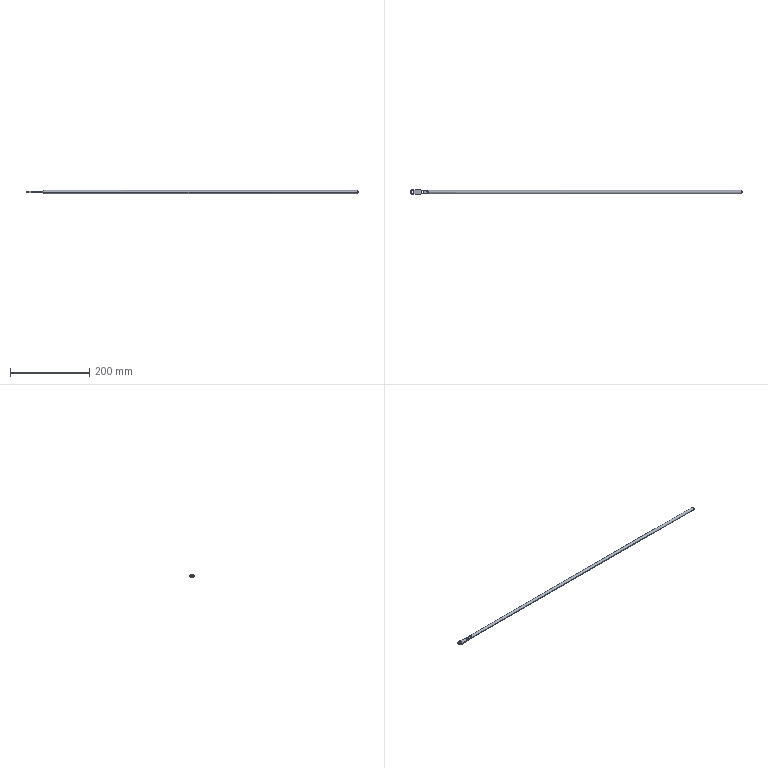Component | SolidWorks | FrontDoorAssembly-1_FrontDoorLowerLockRod-1 | 1 solid | 20 faces | box 837.5 x 13 x 8 mm | volume 41039 mm3 | plane 11 | cylinder 7 | cone 2 | commonest cylinder face diameters 6.5 x4 8 x2 13 x1
build123d program:
from build123d import *

# Parameters (mm, degrees)
SKETCH1_R           = 4
BOSS_EXTRUDE1_DEPTH = 837.5
CUT_EXTRUDE1_DEPTH  = 5
SKETCH3_W           = 42
SKETCH3_H           = 2.024
CUT_EXTRUDE2_DEPTH  = 10
BOSS_EXTRUDE2_DEPTH = 3
CUT_EXTRUDE3_DEPTH  = 3
SKETCH6_R           = 3.25
CUT_EXTRUDE4_DEPTH  = 3
CHAMFER1_SIZE       = 1.5


with BuildPart() as part:
    # Sketch1 → Boss-Extrude1 (new body)
    with BuildSketch(Plane(origin=(0, 0, 0), x_dir=(0, 0, -1), z_dir=(1, 0, 0))):
        Circle(SKETCH1_R)
    extrude(amount=-BOSS_EXTRUDE1_DEPTH)

    # Sketch2 → Cut-Extrude1 (cut, symmetric)
    with BuildSketch(Plane.XY):
        Polygon((-42, 1.5), (-45.678, 4), (-42, 4), (0, 4), (0, 1.5), align=None)
        Polygon((-45.678, -4), (-42, -4), (0, -4), (0, -1.5), (-42, -1.5), align=None)
    extrude(amount=CUT_EXTRUDE1_DEPTH, both=True, mode=Mode.SUBTRACT)

    # Sketch3 → Cut-Extrude2 (cut)
    with BuildSketch(Plane(origin=(0, 1.5, 0), x_dir=(1, 0, 0), z_dir=(0, 1, 0))):
        with Locations((-21, 2.988)):
            Rectangle(SKETCH3_W, SKETCH3_H)
        with Locations((-21, -2.988)):
            Rectangle(SKETCH3_W, SKETCH3_H)
    extrude(amount=-CUT_EXTRUDE2_DEPTH, mode=Mode.SUBTRACT)

    # Sketch4 → Boss-Extrude2 (add)
    with BuildSketch(Plane(origin=(0, 1.5, 0), x_dir=(1, 0, 0), z_dir=(0, 1, 0))):
        with BuildLine():
            Line((-42, -4), (-42, 4))
            Line((-42, 4), (-7.386, 6.439))
            ThreePointArc((-7.386, 6.439), (0, 0), (-7.386, -6.439))
            Line((-7.386, -6.439), (-42, -4))
        make_face()
    extrude(amount=-BOSS_EXTRUDE2_DEPTH)

    # Sketch5 → Cut-Extrude3 (cut)
    with BuildSketch(Plane(origin=(0, 1.5, 0), x_dir=(1, 0, 0), z_dir=(0, 1, 0))):
        with BuildLine():
            Line((-0.8017, 3.127), (2.344, 3.127))
            Line((2.344, 3.127), (2.344, -3.404))
            Line((2.344, -3.404), (-0.9628, -3.404))
            ThreePointArc((-0.9628, -3.404), (-0.001977, -0.1603), (-0.8017, 3.127))
        make_face()
    extrude(amount=-CUT_EXTRUDE3_DEPTH, mode=Mode.SUBTRACT)

    # Sketch6 → Cut-Extrude4 (cut)
    with BuildSketch(Plane(origin=(0, 1.5, 0), x_dir=(1, 0, 0), z_dir=(0, 1, 0))):
        with Locations(Location((-6, 0, 0), (0, 0, 180))):
            Circle(SKETCH6_R)
        with Locations(Location((-31, 0, 0), (0, 0, 180))):
            Circle(SKETCH6_R)
    extrude(amount=-CUT_EXTRUDE4_DEPTH, mode=Mode.SUBTRACT)

    # Chamfer1
    chamfer1_edges = [part.edges().sort_by_distance(p)[0] for p in [
        (-837.5, 0, 4),
    ]]
    chamfer(chamfer1_edges, length=CHAMFER1_SIZE)


solid = part.part

# Placed as in the assembly
solid = solid.moved(Location((30.814, -273.299, 374.754), (-90, 0, 180)))
STEP:
#1=COLOUR_RGB('',0.7922,0.8196,0.9333);
#2=FILL_AREA_STYLE_COLOUR('',#1);
#3=FILL_AREA_STYLE('',(#2));
#4=SURFACE_STYLE_FILL_AREA(#3);
#5=SURFACE_SIDE_STYLE('',(#4));
#6=SURFACE_STYLE_USAGE(.BOTH.,#5);
#7=PRESENTATION_STYLE_ASSIGNMENT((#6));
#8=CARTESIAN_POINT('',(34.186,-10.661,14.754));
#9=VERTEX_POINT('',#8);
#10=CARTESIAN_POINT('',(34.186,-10.858,14.754));
#11=VERTEX_POINT('',#10);
#12=CARTESIAN_POINT('',(34.186,-10.76,14.754));
#13=DIRECTION('',(1.,0.,-0.));
#14=DIRECTION('',(0.,-1.,0.));
#15=AXIS2_PLACEMENT_3D('',#12,#13,#14);
#16=CIRCLE('',#15,0.09843);
#17=EDGE_CURVE('',#9,#11,#16,.T.);
#18=ORIENTED_EDGE('',*,*,#17,.F.);
#19=CARTESIAN_POINT('',(34.127,-10.602,14.754));
#20=VERTEX_POINT('',#19);
#21=CARTESIAN_POINT('',(34.127,-10.602,14.754));
#22=DIRECTION('',(-0.7071,0.7071,0.));
#23=VECTOR('',#22,39.37);
#24=LINE('',#21,#23);
#25=EDGE_CURVE('',#9,#20,#24,.T.);
#26=ORIENTED_EDGE('',*,*,#25,.T.);
#27=CARTESIAN_POINT('',(34.127,-10.917,14.754));
#28=VERTEX_POINT('',#27);
#29=CARTESIAN_POINT('',(34.127,-10.76,14.754));
#30=DIRECTION('',(-1.,-0.,0.));
#31=DIRECTION('',(0.,-1.,0.));
#32=AXIS2_PLACEMENT_3D('',#29,#30,#31);
#33=CIRCLE('',#32,0.1575);
#34=EDGE_CURVE('',#28,#20,#33,.T.);
#35=ORIENTED_EDGE('',*,*,#34,.F.);
#36=CARTESIAN_POINT('',(34.127,-10.917,14.754));
#37=DIRECTION('',(-0.7071,-0.7071,0.));
#38=VECTOR('',#37,39.37);
#39=LINE('',#36,#38);
#40=EDGE_CURVE('',#11,#28,#39,.T.);
#41=ORIENTED_EDGE('',*,*,#40,.F.);
#42=EDGE_LOOP('',(#18,#26,#35,#41));
#43=FACE_OUTER_BOUND('',#42,.T.);
#44=CARTESIAN_POINT('',(34.127,-10.76,14.754));
#45=DIRECTION('',(-1.,-0.,0.));
#46=DIRECTION('',(0.,-1.,0.));
#47=AXIS2_PLACEMENT_3D('',#44,#45,#46);
#48=CONICAL_SURFACE('',#47,0.1575,0.7854);
#49=ADVANCED_FACE('',(#43),#48,.T.);
#50=CARTESIAN_POINT('',(2.306,-10.76,14.695));
#51=VERTEX_POINT('',#50);
#52=CARTESIAN_POINT('',(2.562,-10.76,14.695));
#53=VERTEX_POINT('',#52);
#54=CARTESIAN_POINT('',(2.434,-10.76,14.695));
#55=DIRECTION('',(0.,0.,1.));
#56=DIRECTION('',(1.,0.,0.));
#57=AXIS2_PLACEMENT_3D('',#54,#55,#56);
#58=CIRCLE('',#57,0.128);
#59=EDGE_CURVE('',#51,#53,#58,.T.);
#60=ORIENTED_EDGE('',*,*,#59,.F.);
#61=CARTESIAN_POINT('',(2.306,-10.76,14.813));
#62=VERTEX_POINT('',#61);
#63=CARTESIAN_POINT('',(2.306,-10.76,14.695));
#64=DIRECTION('',(0.,0.,1.));
#65=VECTOR('',#64,39.37);
#66=LINE('',#63,#65);
#67=EDGE_CURVE('',#51,#62,#66,.T.);
#68=ORIENTED_EDGE('',*,*,#67,.T.);
#69=CARTESIAN_POINT('',(2.562,-10.76,14.813));
#70=VERTEX_POINT('',#69);
#71=CARTESIAN_POINT('',(2.434,-10.76,14.813));
#72=DIRECTION('',(0.,0.,1.));
#73=DIRECTION('',(1.,0.,0.));
#74=AXIS2_PLACEMENT_3D('',#71,#72,#73);
#75=CIRCLE('',#74,0.128);
#76=EDGE_CURVE('',#62,#70,#75,.T.);
#77=ORIENTED_EDGE('',*,*,#76,.T.);
#78=CARTESIAN_POINT('',(2.562,-10.76,14.695));
#79=DIRECTION('',(0.,0.,1.));
#80=VECTOR('',#79,39.37);
#81=LINE('',#78,#80);
#82=EDGE_CURVE('',#53,#70,#81,.T.);
#83=ORIENTED_EDGE('',*,*,#82,.F.);
#84=EDGE_LOOP('',(#60,#68,#77,#83));
#85=FACE_OUTER_BOUND('',#84,.T.);
#86=CARTESIAN_POINT('',(2.434,-10.76,14.695));
#87=DIRECTION('',(0.,0.,1.));
#88=DIRECTION('',(1.,0.,0.));
#89=AXIS2_PLACEMENT_3D('',#86,#87,#88);
#90=CYLINDRICAL_SURFACE('',#89,0.128);
#91=ADVANCED_FACE('',(#85),#90,.F.);
#92=CARTESIAN_POINT('',(1.321,-10.76,14.695));
#93=VERTEX_POINT('',#92);
#94=CARTESIAN_POINT('',(1.577,-10.76,14.695));
#95=VERTEX_POINT('',#94);
#96=CARTESIAN_POINT('',(1.449,-10.76,14.695));
#97=DIRECTION('',(0.,0.,1.));
#98=DIRECTION('',(1.,0.,0.));
#99=AXIS2_PLACEMENT_3D('',#96,#97,#98);
#100=CIRCLE('',#99,0.128);
#101=EDGE_CURVE('',#93,#95,#100,.T.);
#102=ORIENTED_EDGE('',*,*,#101,.F.);
#103=CARTESIAN_POINT('',(1.321,-10.76,14.813));
#104=VERTEX_POINT('',#103);
#105=CARTESIAN_POINT('',(1.321,-10.76,14.695));
#106=DIRECTION('',(0.,0.,1.));
#107=VECTOR('',#106,39.37);
#108=LINE('',#105,#107);
#109=EDGE_CURVE('',#93,#104,#108,.T.);
#110=ORIENTED_EDGE('',*,*,#109,.T.);
#111=CARTESIAN_POINT('',(1.577,-10.76,14.813));
#112=VERTEX_POINT('',#111);
#113=CARTESIAN_POINT('',(1.449,-10.76,14.813));
#114=DIRECTION('',(0.,0.,1.));
#115=DIRECTION('',(1.,0.,0.));
#116=AXIS2_PLACEMENT_3D('',#113,#114,#115);
#117=CIRCLE('',#116,0.128);
#118=EDGE_CURVE('',#104,#112,#117,.T.);
#119=ORIENTED_EDGE('',*,*,#118,.T.);
#120=CARTESIAN_POINT('',(1.577,-10.76,14.695));
#121=DIRECTION('',(0.,0.,1.));
#122=VECTOR('',#121,39.37);
#123=LINE('',#120,#122);
#124=EDGE_CURVE('',#95,#112,#123,.T.);
#125=ORIENTED_EDGE('',*,*,#124,.F.);
#126=EDGE_LOOP('',(#102,#110,#119,#125));
#127=FACE_OUTER_BOUND('',#126,.T.);
#128=CARTESIAN_POINT('',(1.449,-10.76,14.695));
#129=DIRECTION('',(0.,0.,1.));
#130=DIRECTION('',(1.,0.,0.));
#131=AXIS2_PLACEMENT_3D('',#128,#129,#130);
#132=CYLINDRICAL_SURFACE('',#131,0.128);
#133=ADVANCED_FACE('',(#127),#132,.F.);
#134=ORIENTED_EDGE('',*,*,#34,.T.);
#135=CARTESIAN_POINT('',(2.867,-10.602,14.754));
#136=VERTEX_POINT('',#135);
#137=CARTESIAN_POINT('',(34.186,-10.602,14.754));
#138=DIRECTION('',(-1.,-0.,0.));
#139=VECTOR('',#138,39.37);
#140=LINE('',#137,#139);
#141=EDGE_CURVE('',#20,#136,#140,.T.);
#142=ORIENTED_EDGE('',*,*,#141,.T.);
#143=CARTESIAN_POINT('',(2.867,-10.614,14.813));
#144=VERTEX_POINT('',#143);
#145=CARTESIAN_POINT('',(2.867,-10.76,14.754));
#146=DIRECTION('',(-1.,-0.,0.));
#147=DIRECTION('',(0.,0.,-1.));
#148=AXIS2_PLACEMENT_3D('',#145,#146,#147);
#149=CIRCLE('',#148,0.1575);
#150=EDGE_CURVE('',#144,#136,#149,.T.);
#151=ORIENTED_EDGE('',*,*,#150,.F.);
#152=CARTESIAN_POINT('',(2.867,-10.906,14.813));
#153=VERTEX_POINT('',#152);
#154=CARTESIAN_POINT('',(2.867,-10.906,14.813));
#155=CARTESIAN_POINT('',(3.094,-10.843,14.968));
#156=CARTESIAN_POINT('',(3.094,-10.676,14.968));
#157=CARTESIAN_POINT('',(2.867,-10.614,14.813));
#158=(BOUNDED_CURVE()B_SPLINE_CURVE(3,(#154,#155,#156,#157),.UNSPECIFIED.,.F.,.F.)B_SPLINE_CURVE_WITH_KNOTS((4,4),(1.955,4.328),.UNSPECIFIED.)CURVE()GEOMETRIC_REPRESENTATION_ITEM()RATIONAL_B_SPLINE_CURVE((1.,0.5833,0.5833,1.))REPRESENTATION_ITEM(''));
#159=EDGE_CURVE('',#153,#144,#158,.T.);
#160=ORIENTED_EDGE('',*,*,#159,.F.);
#161=CARTESIAN_POINT('',(2.867,-10.917,14.754));
#162=VERTEX_POINT('',#161);
#163=CARTESIAN_POINT('',(2.867,-10.76,14.754));
#164=DIRECTION('',(-1.,-0.,0.));
#165=DIRECTION('',(0.,0.,-1.));
#166=AXIS2_PLACEMENT_3D('',#163,#164,#165);
#167=CIRCLE('',#166,0.1575);
#168=EDGE_CURVE('',#162,#153,#167,.T.);
#169=ORIENTED_EDGE('',*,*,#168,.F.);
#170=CARTESIAN_POINT('',(34.186,-10.917,14.754));
#171=DIRECTION('',(-1.,-0.,0.));
#172=VECTOR('',#171,39.37);
#173=LINE('',#170,#172);
#174=EDGE_CURVE('',#28,#162,#173,.T.);
#175=ORIENTED_EDGE('',*,*,#174,.F.);
#176=EDGE_LOOP('',(#134,#142,#151,#160,#169,#175));
#177=FACE_OUTER_BOUND('',#176,.T.);
#178=CARTESIAN_POINT('',(34.186,-10.76,14.754));
#179=DIRECTION('',(-1.,-0.,0.));
#180=DIRECTION('',(0.,-1.,0.));
#181=AXIS2_PLACEMENT_3D('',#178,#179,#180);
#182=CYLINDRICAL_SURFACE('',#181,0.1575);
#183=ADVANCED_FACE('',(#177),#182,.T.);
#184=ORIENTED_EDGE('',*,*,#141,.F.);
#185=CARTESIAN_POINT('',(34.127,-10.76,14.754));
#186=DIRECTION('',(-1.,-0.,0.));
#187=DIRECTION('',(0.,-1.,0.));
#188=AXIS2_PLACEMENT_3D('',#185,#186,#187);
#189=CIRCLE('',#188,0.1575);
#190=EDGE_CURVE('',#20,#28,#189,.T.);
#191=ORIENTED_EDGE('',*,*,#190,.T.);
#192=ORIENTED_EDGE('',*,*,#174,.T.);
#193=CARTESIAN_POINT('',(2.867,-10.906,14.695));
#194=VERTEX_POINT('',#193);
#195=CARTESIAN_POINT('',(2.867,-10.76,14.754));
#196=DIRECTION('',(-1.,-0.,0.));
#197=DIRECTION('',(0.,-0.,-1.));
#198=AXIS2_PLACEMENT_3D('',#195,#196,#197);
#199=CIRCLE('',#198,0.1575);
#200=EDGE_CURVE('',#194,#162,#199,.T.);
#201=ORIENTED_EDGE('',*,*,#200,.F.);
#202=CARTESIAN_POINT('',(2.867,-10.614,14.695));
#203=VERTEX_POINT('',#202);
#204=CARTESIAN_POINT('',(2.867,-10.614,14.695));
#205=CARTESIAN_POINT('',(3.094,-10.676,14.54));
#206=CARTESIAN_POINT('',(3.094,-10.843,14.54));
#207=CARTESIAN_POINT('',(2.867,-10.906,14.695));
#208=(BOUNDED_CURVE()B_SPLINE_CURVE(3,(#204,#205,#206,#207),.UNSPECIFIED.,.F.,.F.)B_SPLINE_CURVE_WITH_KNOTS((4,4),(1.955,4.328),.UNSPECIFIED.)CURVE()GEOMETRIC_REPRESENTATION_ITEM()RATIONAL_B_SPLINE_CURVE((1.,0.5833,0.5833,1.))REPRESENTATION_ITEM(''));
#209=EDGE_CURVE('',#203,#194,#208,.T.);
#210=ORIENTED_EDGE('',*,*,#209,.F.);
#211=CARTESIAN_POINT('',(2.867,-10.76,14.754));
#212=DIRECTION('',(-1.,-0.,0.));
#213=DIRECTION('',(0.,-0.,-1.));
#214=AXIS2_PLACEMENT_3D('',#211,#212,#213);
#215=CIRCLE('',#214,0.1575);
#216=EDGE_CURVE('',#136,#203,#215,.T.);
#217=ORIENTED_EDGE('',*,*,#216,.F.);
#218=EDGE_LOOP('',(#184,#191,#192,#201,#210,#217));
#219=FACE_OUTER_BOUND('',#218,.T.);
#220=CARTESIAN_POINT('',(34.186,-10.76,14.754));
#221=DIRECTION('',(-1.,-0.,0.));
#222=DIRECTION('',(0.,-1.,0.));
#223=AXIS2_PLACEMENT_3D('',#220,#221,#222);
#224=CYLINDRICAL_SURFACE('',#223,0.1575);
#225=ADVANCED_FACE('',(#219),#224,.T.);
#226=CARTESIAN_POINT('',(34.186,-10.76,14.754));
#227=DIRECTION('',(1.,0.,-0.));
#228=DIRECTION('',(0.,-1.,0.));
#229=AXIS2_PLACEMENT_3D('',#226,#227,#228);
#230=CIRCLE('',#229,0.09843);
#231=EDGE_CURVE('',#11,#9,#230,.T.);
#232=ORIENTED_EDGE('',*,*,#231,.T.);
#233=ORIENTED_EDGE('',*,*,#17,.T.);
#234=EDGE_LOOP('',(#232,#233));
#235=FACE_OUTER_BOUND('',#234,.T.);
#236=CARTESIAN_POINT('',(34.186,-10.76,14.754));
#237=DIRECTION('',(-1.,-0.,0.));
#238=DIRECTION('',(0.,-1.,-0.));
#239=AXIS2_PLACEMENT_3D('',#236,#237,#238);
#240=PLANE('',#239);
#241=ADVANCED_FACE('',(#235),#240,.F.);
#242=CARTESIAN_POINT('',(2.434,-10.76,14.813));
#243=DIRECTION('',(0.,0.,1.));
#244=DIRECTION('',(1.,0.,0.));
#245=AXIS2_PLACEMENT_3D('',#242,#243,#244);
#246=CIRCLE('',#245,0.128);
#247=EDGE_CURVE('',#70,#62,#246,.T.);
#248=ORIENTED_EDGE('',*,*,#247,.F.);
#249=ORIENTED_EDGE('',*,*,#76,.F.);
#250=EDGE_LOOP('',(#248,#249));
#251=FACE_BOUND('',#250,.T.);
#252=CARTESIAN_POINT('',(1.449,-10.76,14.813));
#253=DIRECTION('',(0.,0.,1.));
#254=DIRECTION('',(1.,0.,0.));
#255=AXIS2_PLACEMENT_3D('',#252,#253,#254);
#256=CIRCLE('',#255,0.128);
#257=EDGE_CURVE('',#112,#104,#256,.T.);
#258=ORIENTED_EDGE('',*,*,#257,.F.);
#259=ORIENTED_EDGE('',*,*,#118,.F.);
#260=EDGE_LOOP('',(#258,#259));
#261=FACE_BOUND('',#260,.T.);
#262=CARTESIAN_POINT('',(2.867,-10.602,14.813));
#263=VERTEX_POINT('',#262);
#264=CARTESIAN_POINT('',(1.504,-10.506,14.813));
#265=VERTEX_POINT('',#264);
#266=CARTESIAN_POINT('',(2.867,-10.602,14.813));
#267=DIRECTION('',(-0.9975,0.0703,0.));
#268=VECTOR('',#267,39.37);
#269=LINE('',#266,#268);
#270=EDGE_CURVE('',#263,#265,#269,.T.);
#271=ORIENTED_EDGE('',*,*,#270,.T.);
#272=CARTESIAN_POINT('',(1.504,-11.013,14.813));
#273=VERTEX_POINT('',#272);
#274=CARTESIAN_POINT('',(1.469,-10.76,14.813));
#275=DIRECTION('',(0.,0.,1.));
#276=DIRECTION('',(1.,0.,0.));
#277=AXIS2_PLACEMENT_3D('',#274,#275,#276);
#278=CIRCLE('',#277,0.2559);
#279=EDGE_CURVE('',#265,#273,#278,.T.);
#280=ORIENTED_EDGE('',*,*,#279,.T.);
#281=CARTESIAN_POINT('',(2.867,-10.917,14.813));
#282=VERTEX_POINT('',#281);
#283=CARTESIAN_POINT('',(2.867,-10.917,14.813));
#284=DIRECTION('',(0.9975,0.0703,-0.));
#285=VECTOR('',#284,39.37);
#286=LINE('',#283,#285);
#287=EDGE_CURVE('',#273,#282,#286,.T.);
#288=ORIENTED_EDGE('',*,*,#287,.T.);
#289=CARTESIAN_POINT('',(2.867,-10.602,14.813));
#290=DIRECTION('',(-0.,1.,0.));
#291=VECTOR('',#290,39.37);
#292=LINE('',#289,#291);
#293=EDGE_CURVE('',#282,#153,#292,.T.);
#294=ORIENTED_EDGE('',*,*,#293,.T.);
#295=CARTESIAN_POINT('',(2.867,-10.957,14.813));
#296=DIRECTION('',(-0.,1.,0.));
#297=VECTOR('',#296,39.37);
#298=LINE('',#295,#297);
#299=EDGE_CURVE('',#153,#144,#298,.T.);
#300=ORIENTED_EDGE('',*,*,#299,.T.);
#301=CARTESIAN_POINT('',(2.867,-10.602,14.813));
#302=DIRECTION('',(-0.,1.,0.));
#303=VECTOR('',#302,39.37);
#304=LINE('',#301,#303);
#305=EDGE_CURVE('',#144,#263,#304,.T.);
#306=ORIENTED_EDGE('',*,*,#305,.T.);
#307=EDGE_LOOP('',(#271,#280,#288,#294,#300,#306));
#308=FACE_OUTER_BOUND('',#307,.T.);
#309=CARTESIAN_POINT('',(1.213,-10.957,14.813));
#310=DIRECTION('',(-0.,-0.,-1.));
#311=DIRECTION('',(-1.,-0.,0.));
#312=AXIS2_PLACEMENT_3D('',#309,#310,#311);
#313=PLANE('',#312);
#314=ADVANCED_FACE('',(#251,#261,#308),#313,.F.);
#315=ORIENTED_EDGE('',*,*,#299,.F.);
#316=ORIENTED_EDGE('',*,*,#159,.T.);
#317=EDGE_LOOP('',(#315,#316));
#318=FACE_OUTER_BOUND('',#317,.T.);
#319=CARTESIAN_POINT('',(2.867,-10.957,14.813));
#320=DIRECTION('',(0.5621,0.,-0.8271));
#321=DIRECTION('',(-0.8271,-0.,-0.5621));
#322=AXIS2_PLACEMENT_3D('',#319,#320,#321);
#323=PLANE('',#322);
#324=ADVANCED_FACE('',(#318),#323,.F.);
#325=CARTESIAN_POINT('',(2.867,-10.957,14.695));
#326=DIRECTION('',(-0.,1.,0.));
#327=VECTOR('',#326,39.37);
#328=LINE('',#325,#327);
#329=EDGE_CURVE('',#194,#203,#328,.T.);
#330=ORIENTED_EDGE('',*,*,#329,.T.);
#331=ORIENTED_EDGE('',*,*,#209,.T.);
#332=EDGE_LOOP('',(#330,#331));
#333=FACE_OUTER_BOUND('',#332,.T.);
#334=CARTESIAN_POINT('',(2.867,-10.957,14.695));
#335=DIRECTION('',(0.5621,0.,0.8271));
#336=DIRECTION('',(0.8271,0.,-0.5621));
#337=AXIS2_PLACEMENT_3D('',#334,#335,#336);
#338=PLANE('',#337);
#339=ADVANCED_FACE('',(#333),#338,.F.);
#340=CARTESIAN_POINT('',(2.434,-10.76,14.695));
#341=DIRECTION('',(0.,0.,1.));
#342=DIRECTION('',(1.,0.,0.));
#343=AXIS2_PLACEMENT_3D('',#340,#341,#342);
#344=CIRCLE('',#343,0.128);
#345=EDGE_CURVE('',#53,#51,#344,.T.);
#346=ORIENTED_EDGE('',*,*,#345,.T.);
#347=ORIENTED_EDGE('',*,*,#59,.T.);
#348=EDGE_LOOP('',(#346,#347));
#349=FACE_BOUND('',#348,.T.);
#350=CARTESIAN_POINT('',(1.449,-10.76,14.695));
#351=DIRECTION('',(0.,0.,1.));
#352=DIRECTION('',(1.,0.,0.));
#353=AXIS2_PLACEMENT_3D('',#350,#351,#352);
#354=CIRCLE('',#353,0.128);
#355=EDGE_CURVE('',#95,#93,#354,.T.);
#356=ORIENTED_EDGE('',*,*,#355,.T.);
#357=ORIENTED_EDGE('',*,*,#101,.T.);
#358=EDGE_LOOP('',(#356,#357));
#359=FACE_BOUND('',#358,.T.);
#360=CARTESIAN_POINT('',(1.504,-10.506,14.695));
#361=VERTEX_POINT('',#360);
#362=CARTESIAN_POINT('',(1.504,-11.013,14.695));
#363=VERTEX_POINT('',#362);
#364=CARTESIAN_POINT('',(1.469,-10.76,14.695));
#365=DIRECTION('',(0.,0.,1.));
#366=DIRECTION('',(1.,0.,0.));
#367=AXIS2_PLACEMENT_3D('',#364,#365,#366);
#368=CIRCLE('',#367,0.2559);
#369=EDGE_CURVE('',#361,#363,#368,.T.);
#370=ORIENTED_EDGE('',*,*,#369,.F.);
#371=CARTESIAN_POINT('',(2.867,-10.602,14.695));
#372=VERTEX_POINT('',#371);
#373=CARTESIAN_POINT('',(2.867,-10.602,14.695));
#374=DIRECTION('',(-0.9975,0.0703,0.));
#375=VECTOR('',#374,39.37);
#376=LINE('',#373,#375);
#377=EDGE_CURVE('',#372,#361,#376,.T.);
#378=ORIENTED_EDGE('',*,*,#377,.F.);
#379=CARTESIAN_POINT('',(2.867,-10.602,14.695));
#380=DIRECTION('',(-0.,1.,0.));
#381=VECTOR('',#380,39.37);
#382=LINE('',#379,#381);
#383=EDGE_CURVE('',#203,#372,#382,.T.);
#384=ORIENTED_EDGE('',*,*,#383,.F.);
#385=ORIENTED_EDGE('',*,*,#329,.F.);
#386=CARTESIAN_POINT('',(2.867,-10.917,14.695));
#387=VERTEX_POINT('',#386);
#388=CARTESIAN_POINT('',(2.867,-10.602,14.695));
#389=DIRECTION('',(-0.,1.,0.));
#390=VECTOR('',#389,39.37);
#391=LINE('',#388,#390);
#392=EDGE_CURVE('',#387,#194,#391,.T.);
#393=ORIENTED_EDGE('',*,*,#392,.F.);
#394=CARTESIAN_POINT('',(2.867,-10.917,14.695));
#395=DIRECTION('',(0.9975,0.0703,-0.));
#396=VECTOR('',#395,39.37);
#397=LINE('',#394,#396);
#398=EDGE_CURVE('',#363,#387,#397,.T.);
#399=ORIENTED_EDGE('',*,*,#398,.F.);
#400=EDGE_LOOP('',(#370,#378,#384,#385,#393,#399));
#401=FACE_OUTER_BOUND('',#400,.T.);
#402=CARTESIAN_POINT('',(1.213,-10.957,14.695));
#403=DIRECTION('',(0.,-0.,1.));
#404=DIRECTION('',(1.,0.,-0.));
#405=AXIS2_PLACEMENT_3D('',#402,#403,#404);
#406=PLANE('',#405);
#407=ADVANCED_FACE('',(#349,#359,#401),#406,.F.);
#408=ORIENTED_EDGE('',*,*,#270,.F.);
#409=CARTESIAN_POINT('',(2.867,-10.602,14.695));
#410=DIRECTION('',(0.,0.,1.));
#411=VECTOR('',#410,39.37);
#412=LINE('',#409,#411);
#413=EDGE_CURVE('',#136,#263,#412,.T.);
#414=ORIENTED_EDGE('',*,*,#413,.F.);
#415=CARTESIAN_POINT('',(2.867,-10.602,14.695));
#416=DIRECTION('',(0.,0.,1.));
#417=VECTOR('',#416,39.37);
#418=LINE('',#415,#417);
#419=EDGE_CURVE('',#372,#136,#418,.T.);
#420=ORIENTED_EDGE('',*,*,#419,.F.);
#421=ORIENTED_EDGE('',*,*,#377,.T.);
#422=CARTESIAN_POINT('',(1.504,-10.506,14.695));
#423=DIRECTION('',(0.,0.,1.));
#424=VECTOR('',#423,39.37);
#425=LINE('',#422,#424);
#426=EDGE_CURVE('',#361,#265,#425,.T.);
#427=ORIENTED_EDGE('',*,*,#426,.T.);
#428=EDGE_LOOP('',(#408,#414,#420,#421,#427));
#429=FACE_OUTER_BOUND('',#428,.T.);
#430=CARTESIAN_POINT('',(2.867,-10.602,14.695));
#431=DIRECTION('',(0.0703,0.9975,-0.));
#432=DIRECTION('',(-0.9975,0.0703,0.));
#433=AXIS2_PLACEMENT_3D('',#430,#431,#432);
#434=PLANE('',#433);
#435=ADVANCED_FACE('',(#429),#434,.T.);
#436=ORIENTED_EDGE('',*,*,#419,.T.);
#437=ORIENTED_EDGE('',*,*,#216,.T.);
#438=ORIENTED_EDGE('',*,*,#383,.T.);
#439=EDGE_LOOP('',(#436,#437,#438));
#440=FACE_OUTER_BOUND('',#439,.T.);
#441=CARTESIAN_POINT('',(2.867,-10.602,14.695));
#442=DIRECTION('',(1.,0.,-0.));
#443=DIRECTION('',(-0.,-0.,-1.));
#444=AXIS2_PLACEMENT_3D('',#441,#442,#443);
#445=PLANE('',#444);
#446=ADVANCED_FACE('',(#440),#445,.T.);
#447=ORIENTED_EDGE('',*,*,#305,.F.);
#448=ORIENTED_EDGE('',*,*,#150,.T.);
#449=ORIENTED_EDGE('',*,*,#413,.T.);
#450=EDGE_LOOP('',(#447,#448,#449));
#451=FACE_OUTER_BOUND('',#450,.T.);
#452=CARTESIAN_POINT('',(2.867,-10.602,14.695));
#453=DIRECTION('',(1.,0.,-0.));
#454=DIRECTION('',(-0.,-0.,-1.));
#455=AXIS2_PLACEMENT_3D('',#452,#453,#454);
#456=PLANE('',#455);
#457=ADVANCED_FACE('',(#451),#456,.T.);
#458=ORIENTED_EDGE('',*,*,#392,.T.);
#459=ORIENTED_EDGE('',*,*,#200,.T.);
#460=CARTESIAN_POINT('',(2.867,-10.917,14.695));
#461=DIRECTION('',(0.,0.,1.));
#462=VECTOR('',#461,39.37);
#463=LINE('',#460,#462);
#464=EDGE_CURVE('',#387,#162,#463,.T.);
#465=ORIENTED_EDGE('',*,*,#464,.F.);
#466=EDGE_LOOP('',(#458,#459,#465));
#467=FACE_OUTER_BOUND('',#466,.T.);
#468=CARTESIAN_POINT('',(2.867,-10.602,14.695));
#469=DIRECTION('',(1.,0.,-0.));
#470=DIRECTION('',(-0.,-0.,-1.));
#471=AXIS2_PLACEMENT_3D('',#468,#469,#470);
#472=PLANE('',#471);
#473=ADVANCED_FACE('',(#467),#472,.T.);
#474=CARTESIAN_POINT('',(2.867,-10.917,14.695));
#475=DIRECTION('',(0.,0.,1.));
#476=VECTOR('',#475,39.37);
#477=LINE('',#474,#476);
#478=EDGE_CURVE('',#162,#282,#477,.T.);
#479=ORIENTED_EDGE('',*,*,#478,.F.);
#480=ORIENTED_EDGE('',*,*,#168,.T.);
#481=ORIENTED_EDGE('',*,*,#293,.F.);
#482=EDGE_LOOP('',(#479,#480,#481));
#483=FACE_OUTER_BOUND('',#482,.T.);
#484=CARTESIAN_POINT('',(2.867,-10.602,14.695));
#485=DIRECTION('',(1.,0.,-0.));
#486=DIRECTION('',(-0.,-0.,-1.));
#487=AXIS2_PLACEMENT_3D('',#484,#485,#486);
#488=PLANE('',#487);
#489=ADVANCED_FACE('',(#483),#488,.T.);
#490=CARTESIAN_POINT('',(1.504,-11.013,14.695));
#491=DIRECTION('',(0.,0.,1.));
#492=VECTOR('',#491,39.37);
#493=LINE('',#490,#492);
#494=EDGE_CURVE('',#363,#273,#493,.T.);
#495=ORIENTED_EDGE('',*,*,#494,.T.);
#496=ORIENTED_EDGE('',*,*,#279,.F.);
#497=ORIENTED_EDGE('',*,*,#426,.F.);
#498=ORIENTED_EDGE('',*,*,#369,.T.);
#499=EDGE_LOOP('',(#495,#496,#497,#498));
#500=FACE_OUTER_BOUND('',#499,.T.);
#501=CARTESIAN_POINT('',(1.469,-10.76,14.695));
#502=DIRECTION('',(0.,0.,1.));
#503=DIRECTION('',(1.,0.,0.));
#504=AXIS2_PLACEMENT_3D('',#501,#502,#503);
#505=CYLINDRICAL_SURFACE('',#504,0.2559);
#506=ADVANCED_FACE('',(#500),#505,.T.);
#507=ORIENTED_EDGE('',*,*,#287,.F.);
#508=ORIENTED_EDGE('',*,*,#494,.F.);
#509=ORIENTED_EDGE('',*,*,#398,.T.);
#510=ORIENTED_EDGE('',*,*,#464,.T.);
#511=ORIENTED_EDGE('',*,*,#478,.T.);
#512=EDGE_LOOP('',(#507,#508,#509,#510,#511));
#513=FACE_OUTER_BOUND('',#512,.T.);
#514=CARTESIAN_POINT('',(2.867,-10.917,14.695));
#515=DIRECTION('',(0.0703,-0.9975,-0.));
#516=DIRECTION('',(0.9975,0.0703,-0.));
#517=AXIS2_PLACEMENT_3D('',#514,#515,#516);
#518=PLANE('',#517);
#519=ADVANCED_FACE('',(#513),#518,.T.);
#520=ORIENTED_EDGE('',*,*,#109,.F.);
#521=ORIENTED_EDGE('',*,*,#355,.F.);
#522=ORIENTED_EDGE('',*,*,#124,.T.);
#523=ORIENTED_EDGE('',*,*,#257,.T.);
#524=EDGE_LOOP('',(#520,#521,#522,#523));
#525=FACE_OUTER_BOUND('',#524,.T.);
#526=CARTESIAN_POINT('',(1.449,-10.76,14.695));
#527=DIRECTION('',(0.,0.,1.));
#528=DIRECTION('',(1.,0.,0.));
#529=AXIS2_PLACEMENT_3D('',#526,#527,#528);
#530=CYLINDRICAL_SURFACE('',#529,0.128);
#531=ADVANCED_FACE('',(#525),#530,.F.);
#532=ORIENTED_EDGE('',*,*,#67,.F.);
#533=ORIENTED_EDGE('',*,*,#345,.F.);
#534=ORIENTED_EDGE('',*,*,#82,.T.);
#535=ORIENTED_EDGE('',*,*,#247,.T.);
#536=EDGE_LOOP('',(#532,#533,#534,#535));
#537=FACE_OUTER_BOUND('',#536,.T.);
#538=CARTESIAN_POINT('',(2.434,-10.76,14.695));
#539=DIRECTION('',(0.,0.,1.));
#540=DIRECTION('',(1.,0.,0.));
#541=AXIS2_PLACEMENT_3D('',#538,#539,#540);
#542=CYLINDRICAL_SURFACE('',#541,0.128);
#543=ADVANCED_FACE('',(#537),#542,.F.);
#544=ORIENTED_EDGE('',*,*,#25,.F.);
#545=ORIENTED_EDGE('',*,*,#231,.F.);
#546=ORIENTED_EDGE('',*,*,#40,.T.);
#547=ORIENTED_EDGE('',*,*,#190,.F.);
#548=EDGE_LOOP('',(#544,#545,#546,#547));
#549=FACE_OUTER_BOUND('',#548,.T.);
#550=CARTESIAN_POINT('',(34.127,-10.76,14.754));
#551=DIRECTION('',(-1.,-0.,0.));
#552=DIRECTION('',(0.,-1.,0.));
#553=AXIS2_PLACEMENT_3D('',#550,#551,#552);
#554=CONICAL_SURFACE('',#553,0.1575,0.7854);
#555=ADVANCED_FACE('',(#549),#554,.T.);
#556=CLOSED_SHELL('',(#49,#91,#133,#183,#225,#241,#314,#324,#339,#407,#435,#446,#457,#473,#489,#506,#519,#531,#543,#555));
#557=MANIFOLD_SOLID_BREP('',#556);
#558=STYLED_ITEM('',(#7),#557);
#559=PRESENTATION_LAYER_ASSIGNMENT('','',(#558));
#560=CARTESIAN_POINT('',(0.,0.,0.));
#561=DIRECTION('',(0.,0.,1.));
#562=DIRECTION('',(1.,0.,0.));
#563=AXIS2_PLACEMENT_3D('',#560,#561,#562);
#564=(LENGTH_UNIT()NAMED_UNIT(*)SI_UNIT($,.METRE.));
#565=LENGTH_MEASURE_WITH_UNIT(LENGTH_MEASURE(0.0254),#564);
#566=DIMENSIONAL_EXPONENTS(1.,0.,0.,0.,0.,0.,0.);
#567=(CONVERSION_BASED_UNIT('',#565)LENGTH_UNIT()NAMED_UNIT(#566));
#568=UNCERTAINTY_MEASURE_WITH_UNIT(LENGTH_MEASURE(0.00001),#567,'','');
#569=(NAMED_UNIT(*)PLANE_ANGLE_UNIT()SI_UNIT($,.RADIAN.));
#570=(NAMED_UNIT(*)SI_UNIT($,.STERADIAN.)SOLID_ANGLE_UNIT());
#571=(GEOMETRIC_REPRESENTATION_CONTEXT(3)GLOBAL_UNCERTAINTY_ASSIGNED_CONTEXT((#568))GLOBAL_UNIT_ASSIGNED_CONTEXT((#567,#569,#570))REPRESENTATION_CONTEXT('',''));
#572=ADVANCED_BREP_SHAPE_REPRESENTATION('',(#557,#563),#571);
#573=(LENGTH_UNIT()NAMED_UNIT(*)SI_UNIT($,.METRE.));
#574=LENGTH_MEASURE_WITH_UNIT(LENGTH_MEASURE(0.0254),#573);
#575=DIMENSIONAL_EXPONENTS(1.,0.,0.,0.,0.,0.,0.);
#576=(CONVERSION_BASED_UNIT('',#574)LENGTH_UNIT()NAMED_UNIT(#575));
#577=UNCERTAINTY_MEASURE_WITH_UNIT(LENGTH_MEASURE(0.00001),#576,'','');
#578=(NAMED_UNIT(*)PLANE_ANGLE_UNIT()SI_UNIT($,.RADIAN.));
#579=(NAMED_UNIT(*)SI_UNIT($,.STERADIAN.)SOLID_ANGLE_UNIT());
#580=(GEOMETRIC_REPRESENTATION_CONTEXT(3)GLOBAL_UNCERTAINTY_ASSIGNED_CONTEXT((#577))GLOBAL_UNIT_ASSIGNED_CONTEXT((#576,#578,#579))REPRESENTATION_CONTEXT('',''));
#581=MECHANICAL_DESIGN_GEOMETRIC_PRESENTATION_REPRESENTATION('',(#558),#580);